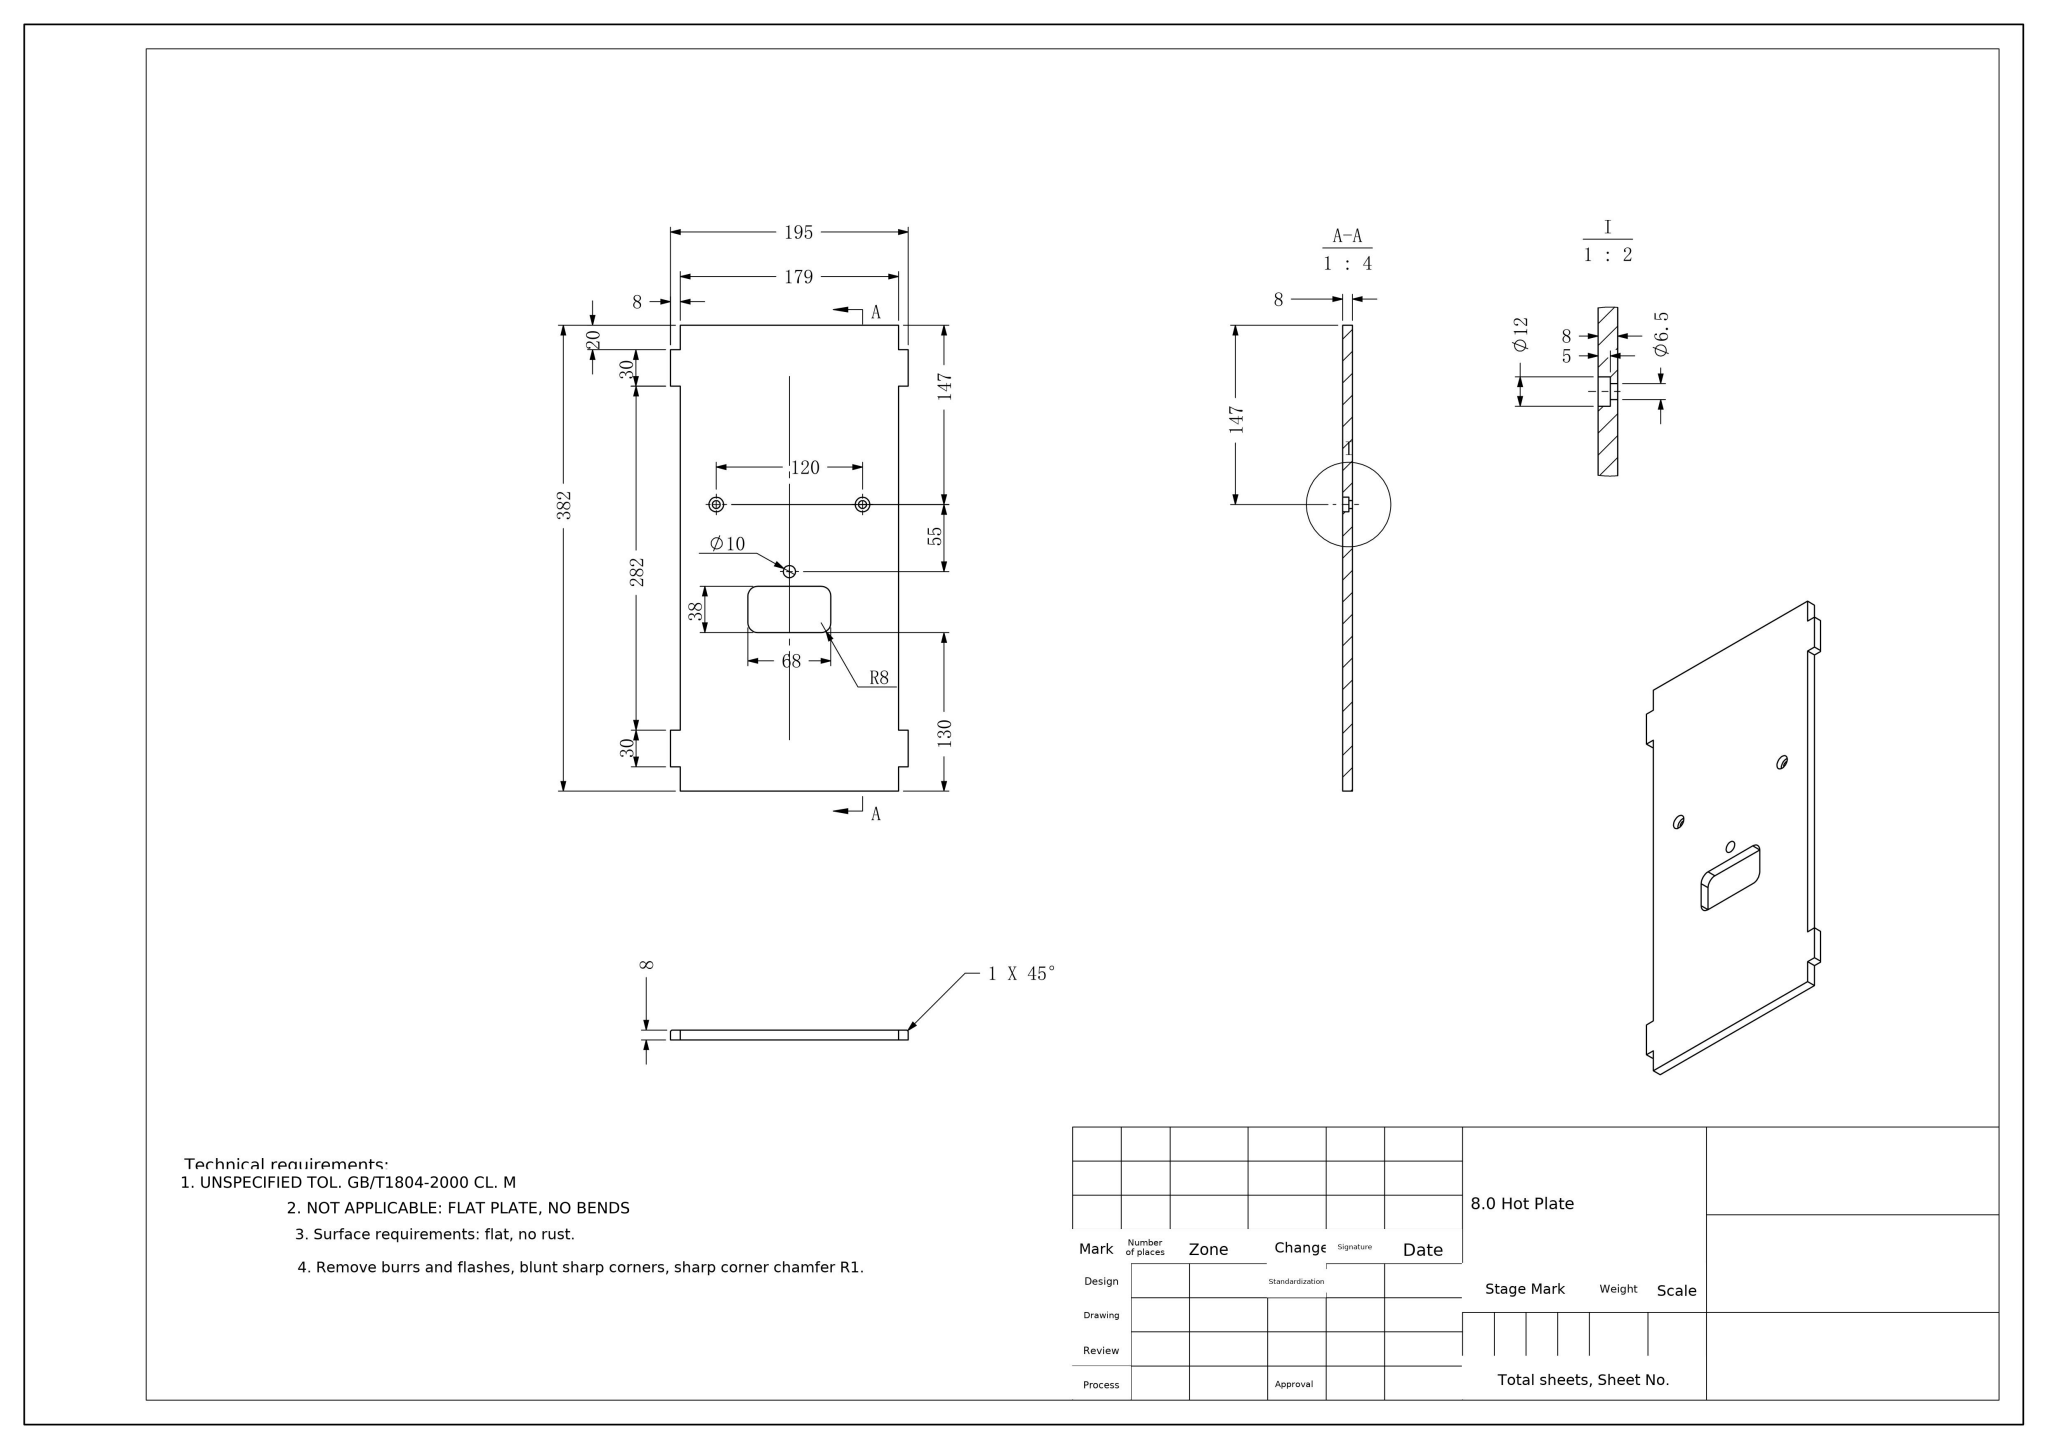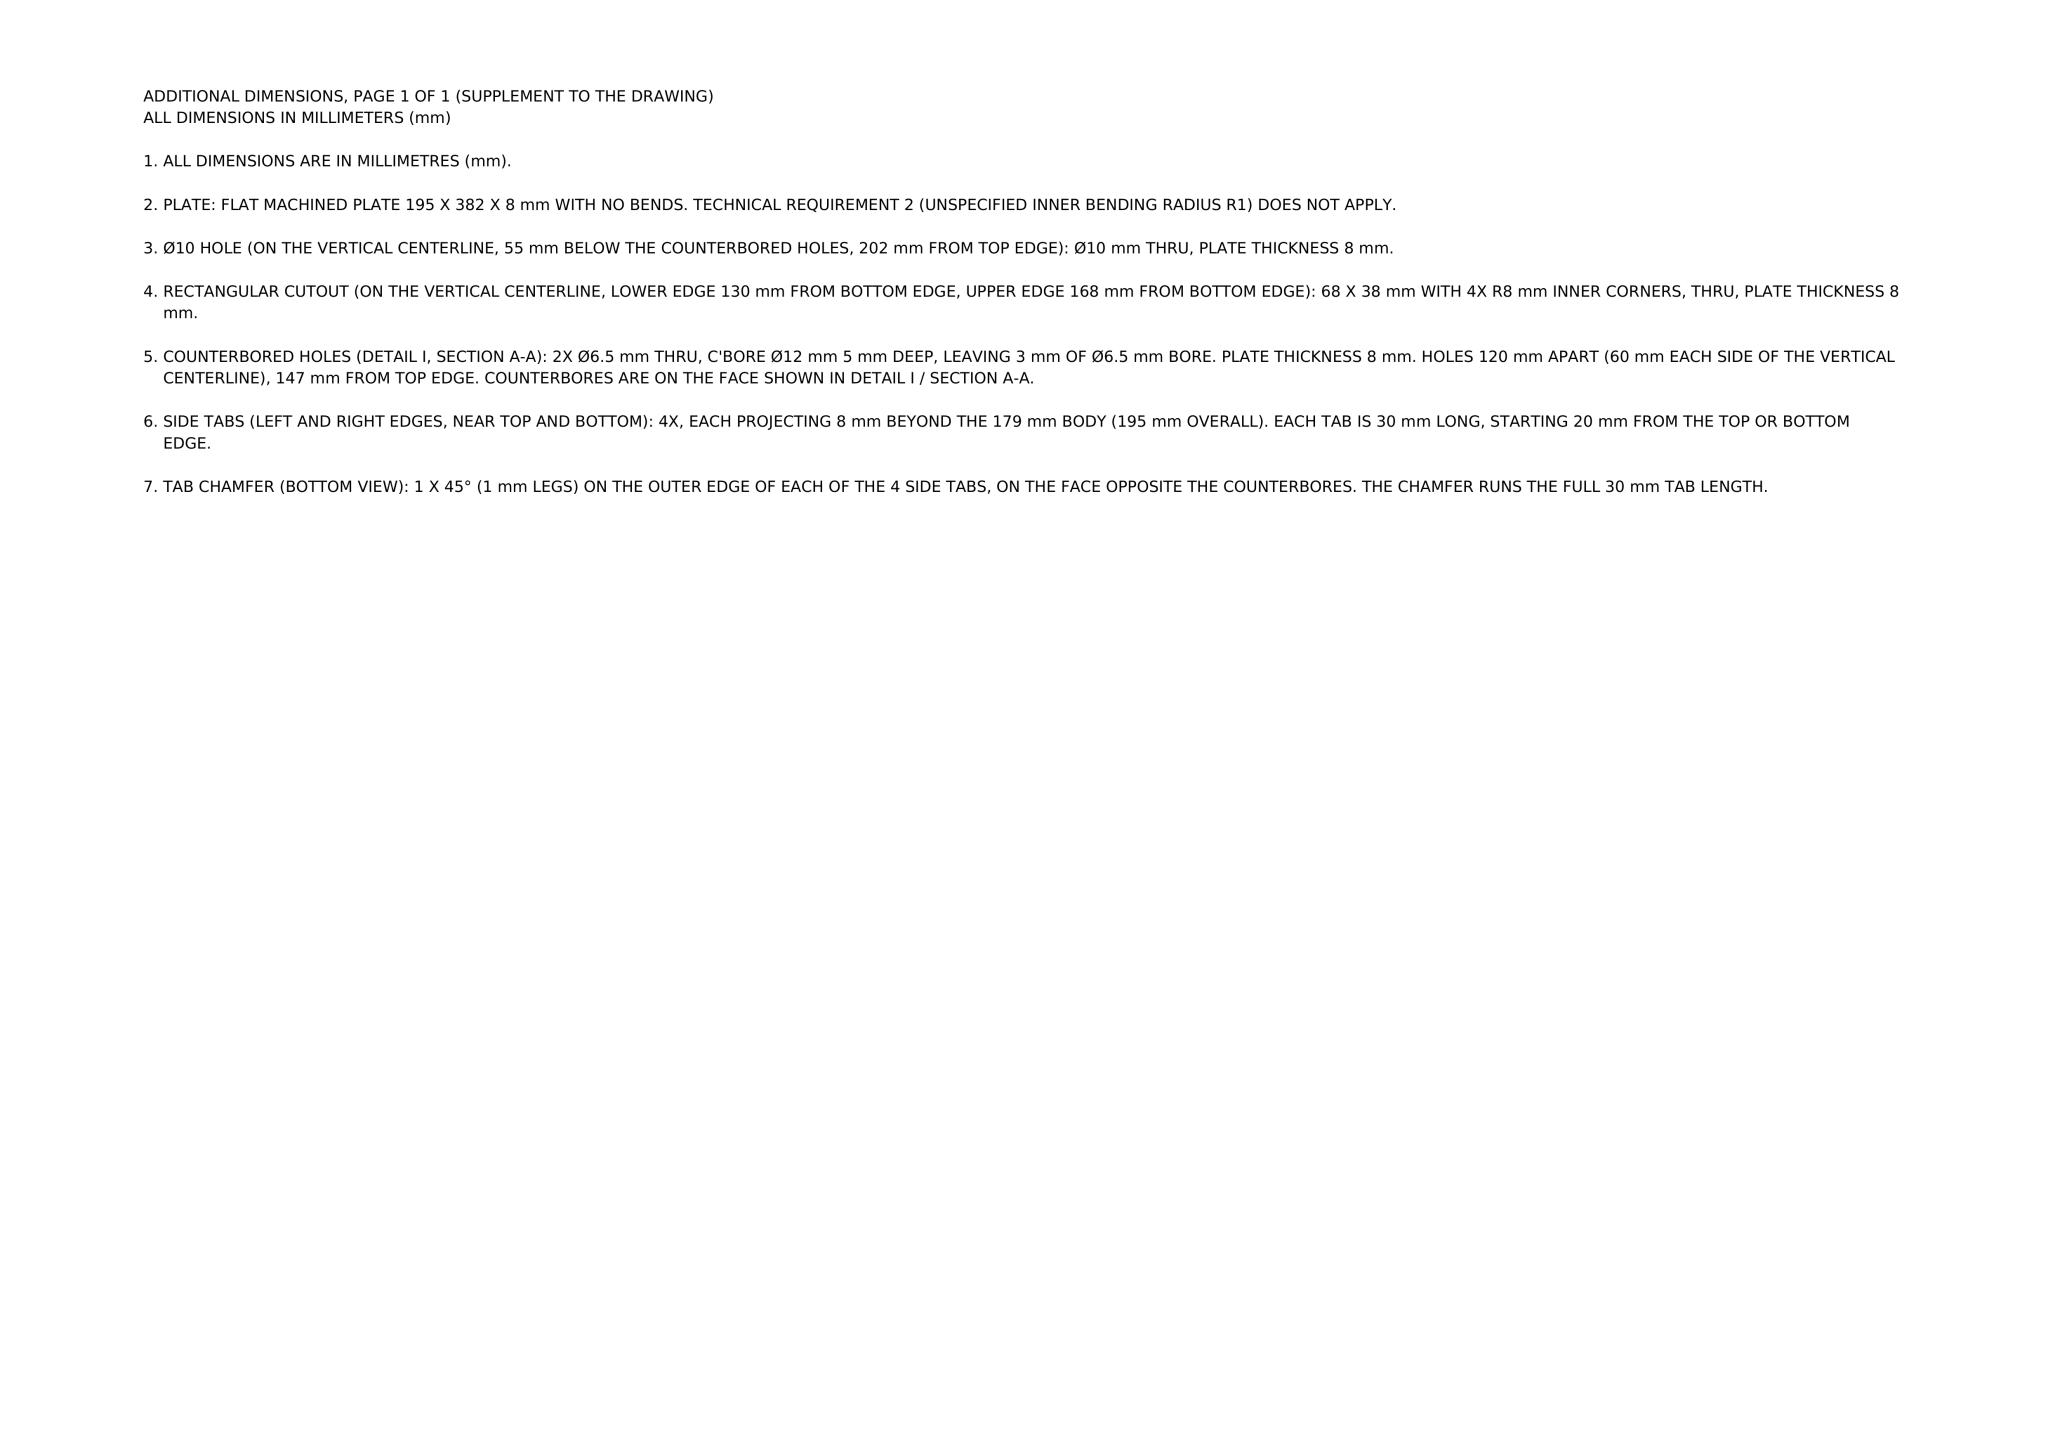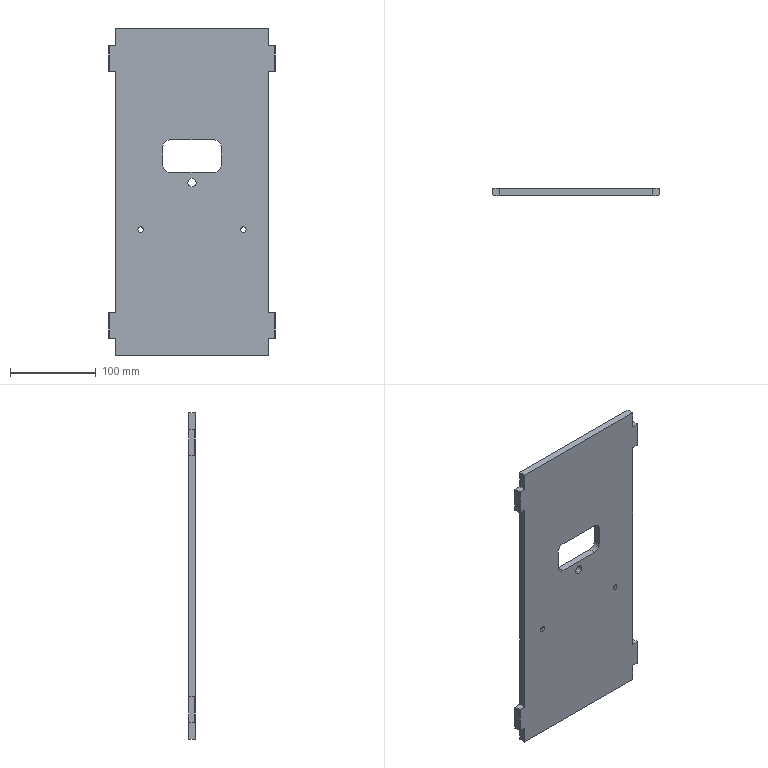Part | NX | mm | 1 solid | 46 faces | box 195 x 8 x 382 mm | volume 532453 mm3 | plane 32 | cylinder 14 | commonest cylinder face diameters 12 x4 6.5 x4 16 x4 10 x2